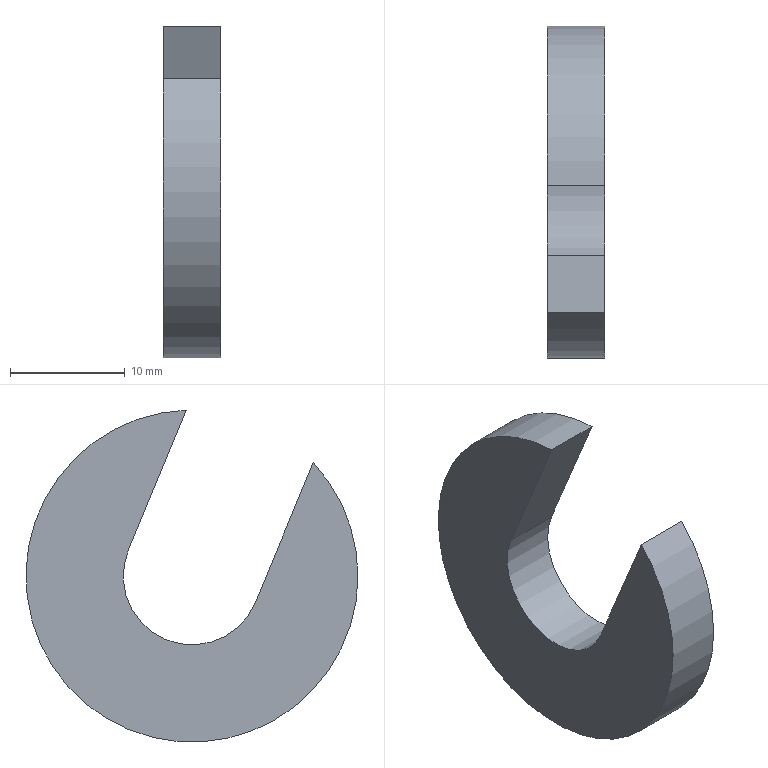Component | NX | WASHER | 1 solid | 6 faces | box 5 x 29 x 28.99 mm | volume 2175 mm3 | plane 4 | cylinder 2 | commonest cylinder face diameters 29 x1 12 x1
STEP:
#1=CARTESIAN_POINT('',(0.,0.,0.));
#2=DIRECTION('',(0.,0.,1.));
#3=DIRECTION('',(1.,0.,0.));
#4=AXIS2_PLACEMENT_3D('',#1,#2,#3);
#5=CARTESIAN_POINT('',(40.592,68.075,199.554));
#6=VERTEX_POINT('',#5);
#7=CARTESIAN_POINT('',(40.592,63.035,211.754));
#8=VERTEX_POINT('',#7);
#9=CARTESIAN_POINT('',(40.592,68.075,199.554));
#10=DIRECTION('',(0.,-0.3818,0.9242));
#11=VECTOR('',#10,1.);
#12=LINE('',#9,#11);
#13=CARTESIAN_POINT('',(45.592,68.075,199.554));
#14=DIRECTION('',(0.,-0.9242,-0.3818));
#15=DIRECTION('',(1.,0.,0.));
#16=AXIS2_PLACEMENT_3D('',#13,#14,#15);
#17=PLANE('',#16);
#18=CARTESIAN_POINT('',(-5.,0.));
#19=DIRECTION('',(0.,1.));
#20=VECTOR('',#19,1.);
#21=LINE('',#18,#20);
#22=(GEOMETRIC_REPRESENTATION_CONTEXT(2)PARAMETRIC_REPRESENTATION_CONTEXT()REPRESENTATION_CONTEXT('',''));
#23=DEFINITIONAL_REPRESENTATION('',(#21),#22);
#24=PCURVE('',#17,#23);
#25=CARTESIAN_POINT('',(40.592,73.621,201.845));
#26=DIRECTION('',(1.,0.,0.));
#27=DIRECTION('',(0.,0.9242,0.3818));
#28=AXIS2_PLACEMENT_3D('',#25,#26,#27);
#29=PLANE('',#28);
#30=CARTESIAN_POINT('',(-6.,-0.));
#31=DIRECTION('',(0.,1.));
#32=VECTOR('',#31,1.);
#33=LINE('',#30,#32);
#34=(GEOMETRIC_REPRESENTATION_CONTEXT(2)PARAMETRIC_REPRESENTATION_CONTEXT()REPRESENTATION_CONTEXT('',''));
#35=DEFINITIONAL_REPRESENTATION('',(#33),#34);
#36=PCURVE('',#29,#35);
#37=SURFACE_CURVE('',#12,(#24,#36),.PCURVE_S1.);
#38=EDGE_CURVE('',#6,#8,#37,.T.);
#39=ORIENTED_EDGE('',*,*,#38,.T.);
#40=CARTESIAN_POINT('',(45.592,63.035,211.754));
#41=VERTEX_POINT('',#40);
#42=CARTESIAN_POINT('',(45.592,63.035,211.754));
#43=DIRECTION('',(-1.,0.,0.));
#44=VECTOR('',#43,1.);
#45=LINE('',#42,#44);
#46=CARTESIAN_POINT('',(0.,13.2));
#47=DIRECTION('',(-1.,0.));
#48=VECTOR('',#47,1.);
#49=LINE('',#46,#48);
#50=(GEOMETRIC_REPRESENTATION_CONTEXT(2)PARAMETRIC_REPRESENTATION_CONTEXT()REPRESENTATION_CONTEXT('',''));
#51=DEFINITIONAL_REPRESENTATION('',(#49),#50);
#52=PCURVE('',#17,#51);
#53=CARTESIAN_POINT('',(45.592,73.621,201.845));
#54=DIRECTION('',(-1.,0.,0.));
#55=DIRECTION('',(0.,-0.9242,-0.3818));
#56=AXIS2_PLACEMENT_3D('',#53,#54,#55);
#57=CYLINDRICAL_SURFACE('',#56,14.5);
#58=CARTESIAN_POINT('',(7.427,0.));
#59=DIRECTION('',(0.,1.));
#60=VECTOR('',#59,1.);
#61=LINE('',#58,#60);
#62=(GEOMETRIC_REPRESENTATION_CONTEXT(2)PARAMETRIC_REPRESENTATION_CONTEXT()REPRESENTATION_CONTEXT('',''));
#63=DEFINITIONAL_REPRESENTATION('',(#61),#62);
#64=PCURVE('',#57,#63);
#65=SURFACE_CURVE('',#45,(#52,#64),.PCURVE_S1.);
#66=EDGE_CURVE('',#41,#8,#65,.T.);
#67=ORIENTED_EDGE('',*,*,#66,.F.);
#68=CARTESIAN_POINT('',(45.592,68.075,199.554));
#69=VERTEX_POINT('',#68);
#70=CARTESIAN_POINT('',(45.592,68.075,199.554));
#71=DIRECTION('',(0.,-0.3818,0.9242));
#72=VECTOR('',#71,1.);
#73=LINE('',#70,#72);
#74=CARTESIAN_POINT('',(0.,0.));
#75=DIRECTION('',(0.,1.));
#76=VECTOR('',#75,1.);
#77=LINE('',#74,#76);
#78=(GEOMETRIC_REPRESENTATION_CONTEXT(2)PARAMETRIC_REPRESENTATION_CONTEXT()REPRESENTATION_CONTEXT('',''));
#79=DEFINITIONAL_REPRESENTATION('',(#77),#78);
#80=PCURVE('',#17,#79);
#81=CARTESIAN_POINT('',(45.592,73.621,201.845));
#82=DIRECTION('',(1.,0.,0.));
#83=DIRECTION('',(0.,0.9242,0.3818));
#84=AXIS2_PLACEMENT_3D('',#81,#82,#83);
#85=PLANE('',#84);
#86=CARTESIAN_POINT('',(-6.,-0.));
#87=DIRECTION('',(0.,1.));
#88=VECTOR('',#87,1.);
#89=LINE('',#86,#88);
#90=(GEOMETRIC_REPRESENTATION_CONTEXT(2)PARAMETRIC_REPRESENTATION_CONTEXT()REPRESENTATION_CONTEXT('',''));
#91=DEFINITIONAL_REPRESENTATION('',(#89),#90);
#92=PCURVE('',#85,#91);
#93=SURFACE_CURVE('',#73,(#80,#92),.PCURVE_S1.);
#94=EDGE_CURVE('',#69,#41,#93,.T.);
#95=ORIENTED_EDGE('',*,*,#94,.F.);
#96=CARTESIAN_POINT('',(45.592,68.075,199.554));
#97=DIRECTION('',(-1.,0.,0.));
#98=VECTOR('',#97,1.);
#99=LINE('',#96,#98);
#100=CARTESIAN_POINT('',(0.,0.));
#101=DIRECTION('',(-1.,0.));
#102=VECTOR('',#101,1.);
#103=LINE('',#100,#102);
#104=(GEOMETRIC_REPRESENTATION_CONTEXT(2)PARAMETRIC_REPRESENTATION_CONTEXT()REPRESENTATION_CONTEXT('',''));
#105=DEFINITIONAL_REPRESENTATION('',(#103),#104);
#106=PCURVE('',#17,#105);
#107=CARTESIAN_POINT('',(45.592,73.621,201.845));
#108=DIRECTION('',(-1.,0.,0.));
#109=DIRECTION('',(0.,-0.9242,-0.3818));
#110=AXIS2_PLACEMENT_3D('',#107,#108,#109);
#111=CYLINDRICAL_SURFACE('',#110,6.);
#112=CARTESIAN_POINT('',(6.283,0.));
#113=DIRECTION('',(0.,1.));
#114=VECTOR('',#113,1.);
#115=LINE('',#112,#114);
#116=(GEOMETRIC_REPRESENTATION_CONTEXT(2)PARAMETRIC_REPRESENTATION_CONTEXT()REPRESENTATION_CONTEXT('',''));
#117=DEFINITIONAL_REPRESENTATION('',(#115),#116);
#118=PCURVE('',#111,#117);
#119=SURFACE_CURVE('',#99,(#106,#118),.PCURVE_S1.);
#120=EDGE_CURVE('',#69,#6,#119,.T.);
#121=ORIENTED_EDGE('',*,*,#120,.T.);
#122=EDGE_LOOP('',(#39,#67,#95,#121));
#123=FACE_BOUND('',#122,.T.);
#124=ADVANCED_FACE('',(#123),#17,.F.);
#125=CARTESIAN_POINT('',(40.592,74.125,216.336));
#126=VERTEX_POINT('',#125);
#127=CARTESIAN_POINT('',(40.592,73.621,201.845));
#128=DIRECTION('',(1.,0.,0.));
#129=DIRECTION('',(0.,0.9242,0.3818));
#130=AXIS2_PLACEMENT_3D('',#127,#128,#129);
#131=CIRCLE('',#130,14.5);
#132=CARTESIAN_POINT('',(9.425,5.));
#133=DIRECTION('',(-1.,0.));
#134=VECTOR('',#133,1.);
#135=LINE('',#132,#134);
#136=(GEOMETRIC_REPRESENTATION_CONTEXT(2)PARAMETRIC_REPRESENTATION_CONTEXT()REPRESENTATION_CONTEXT('',''));
#137=DEFINITIONAL_REPRESENTATION('',(#135),#136);
#138=PCURVE('',#57,#137);
#139=CARTESIAN_POINT('',(0.,0.));
#140=DIRECTION('',(1.,-0.));
#141=AXIS2_PLACEMENT_2D('',#139,#140);
#142=CIRCLE('',#141,14.5);
#143=(GEOMETRIC_REPRESENTATION_CONTEXT(2)PARAMETRIC_REPRESENTATION_CONTEXT()REPRESENTATION_CONTEXT('',''));
#144=DEFINITIONAL_REPRESENTATION('',(#142),#143);
#145=PCURVE('',#29,#144);
#146=SURFACE_CURVE('',#131,(#138,#145),.PCURVE_S1.);
#147=EDGE_CURVE('',#8,#126,#146,.T.);
#148=ORIENTED_EDGE('',*,*,#147,.T.);
#149=CARTESIAN_POINT('',(45.592,74.125,216.336));
#150=VERTEX_POINT('',#149);
#151=CARTESIAN_POINT('',(45.592,74.125,216.336));
#152=DIRECTION('',(-1.,0.,0.));
#153=VECTOR('',#152,1.);
#154=LINE('',#151,#153);
#155=CARTESIAN_POINT('',(1.997,0.));
#156=DIRECTION('',(0.,1.));
#157=VECTOR('',#156,1.);
#158=LINE('',#155,#157);
#159=(GEOMETRIC_REPRESENTATION_CONTEXT(2)PARAMETRIC_REPRESENTATION_CONTEXT()REPRESENTATION_CONTEXT('',''));
#160=DEFINITIONAL_REPRESENTATION('',(#158),#159);
#161=PCURVE('',#57,#160);
#162=CARTESIAN_POINT('',(45.592,74.125,216.336));
#163=DIRECTION('',(0.,0.9242,0.3818));
#164=DIRECTION('',(-1.,0.,0.));
#165=AXIS2_PLACEMENT_3D('',#162,#163,#164);
#166=PLANE('',#165);
#167=CARTESIAN_POINT('',(0.,0.));
#168=DIRECTION('',(1.,0.));
#169=VECTOR('',#168,1.);
#170=LINE('',#167,#169);
#171=(GEOMETRIC_REPRESENTATION_CONTEXT(2)PARAMETRIC_REPRESENTATION_CONTEXT()REPRESENTATION_CONTEXT('',''));
#172=DEFINITIONAL_REPRESENTATION('',(#170),#171);
#173=PCURVE('',#166,#172);
#174=SURFACE_CURVE('',#154,(#161,#173),.PCURVE_S1.);
#175=EDGE_CURVE('',#150,#126,#174,.T.);
#176=ORIENTED_EDGE('',*,*,#175,.F.);
#177=CARTESIAN_POINT('',(45.592,73.621,201.845));
#178=DIRECTION('',(1.,0.,0.));
#179=DIRECTION('',(0.,0.9242,0.3818));
#180=AXIS2_PLACEMENT_3D('',#177,#178,#179);
#181=CIRCLE('',#180,14.5);
#182=CARTESIAN_POINT('',(9.425,0.));
#183=DIRECTION('',(-1.,0.));
#184=VECTOR('',#183,1.);
#185=LINE('',#182,#184);
#186=(GEOMETRIC_REPRESENTATION_CONTEXT(2)PARAMETRIC_REPRESENTATION_CONTEXT()REPRESENTATION_CONTEXT('',''));
#187=DEFINITIONAL_REPRESENTATION('',(#185),#186);
#188=PCURVE('',#57,#187);
#189=CARTESIAN_POINT('',(0.,0.));
#190=DIRECTION('',(1.,-0.));
#191=AXIS2_PLACEMENT_2D('',#189,#190);
#192=CIRCLE('',#191,14.5);
#193=(GEOMETRIC_REPRESENTATION_CONTEXT(2)PARAMETRIC_REPRESENTATION_CONTEXT()REPRESENTATION_CONTEXT('',''));
#194=DEFINITIONAL_REPRESENTATION('',(#192),#193);
#195=PCURVE('',#85,#194);
#196=SURFACE_CURVE('',#181,(#188,#195),.PCURVE_S1.);
#197=EDGE_CURVE('',#41,#150,#196,.T.);
#198=ORIENTED_EDGE('',*,*,#197,.F.);
#199=ORIENTED_EDGE('',*,*,#66,.T.);
#200=EDGE_LOOP('',(#148,#176,#198,#199));
#201=FACE_BOUND('',#200,.T.);
#202=ADVANCED_FACE('',(#201),#57,.T.);
#203=CARTESIAN_POINT('',(40.592,79.166,204.136));
#204=VERTEX_POINT('',#203);
#205=CARTESIAN_POINT('',(40.592,74.125,216.336));
#206=DIRECTION('',(0.,0.3818,-0.9242));
#207=VECTOR('',#206,1.);
#208=LINE('',#205,#207);
#209=CARTESIAN_POINT('',(5.,0.));
#210=DIRECTION('',(0.,-1.));
#211=VECTOR('',#210,1.);
#212=LINE('',#209,#211);
#213=(GEOMETRIC_REPRESENTATION_CONTEXT(2)PARAMETRIC_REPRESENTATION_CONTEXT()REPRESENTATION_CONTEXT('',''));
#214=DEFINITIONAL_REPRESENTATION('',(#212),#213);
#215=PCURVE('',#166,#214);
#216=CARTESIAN_POINT('',(6.,13.2));
#217=DIRECTION('',(-0.,-1.));
#218=VECTOR('',#217,1.);
#219=LINE('',#216,#218);
#220=(GEOMETRIC_REPRESENTATION_CONTEXT(2)PARAMETRIC_REPRESENTATION_CONTEXT()REPRESENTATION_CONTEXT('',''));
#221=DEFINITIONAL_REPRESENTATION('',(#219),#220);
#222=PCURVE('',#29,#221);
#223=SURFACE_CURVE('',#208,(#215,#222),.PCURVE_S1.);
#224=EDGE_CURVE('',#126,#204,#223,.T.);
#225=ORIENTED_EDGE('',*,*,#224,.T.);
#226=CARTESIAN_POINT('',(45.592,79.166,204.136));
#227=VERTEX_POINT('',#226);
#228=CARTESIAN_POINT('',(45.592,79.166,204.136));
#229=DIRECTION('',(-1.,0.,0.));
#230=VECTOR('',#229,1.);
#231=LINE('',#228,#230);
#232=CARTESIAN_POINT('',(0.,-13.2));
#233=DIRECTION('',(1.,0.));
#234=VECTOR('',#233,1.);
#235=LINE('',#232,#234);
#236=(GEOMETRIC_REPRESENTATION_CONTEXT(2)PARAMETRIC_REPRESENTATION_CONTEXT()REPRESENTATION_CONTEXT('',''));
#237=DEFINITIONAL_REPRESENTATION('',(#235),#236);
#238=PCURVE('',#166,#237);
#239=CARTESIAN_POINT('',(3.142,0.));
#240=DIRECTION('',(0.,1.));
#241=VECTOR('',#240,1.);
#242=LINE('',#239,#241);
#243=(GEOMETRIC_REPRESENTATION_CONTEXT(2)PARAMETRIC_REPRESENTATION_CONTEXT()REPRESENTATION_CONTEXT('',''));
#244=DEFINITIONAL_REPRESENTATION('',(#242),#243);
#245=PCURVE('',#111,#244);
#246=SURFACE_CURVE('',#231,(#238,#245),.PCURVE_S1.);
#247=EDGE_CURVE('',#227,#204,#246,.T.);
#248=ORIENTED_EDGE('',*,*,#247,.F.);
#249=CARTESIAN_POINT('',(45.592,74.125,216.336));
#250=DIRECTION('',(0.,0.3818,-0.9242));
#251=VECTOR('',#250,1.);
#252=LINE('',#249,#251);
#253=CARTESIAN_POINT('',(0.,0.));
#254=DIRECTION('',(0.,-1.));
#255=VECTOR('',#254,1.);
#256=LINE('',#253,#255);
#257=(GEOMETRIC_REPRESENTATION_CONTEXT(2)PARAMETRIC_REPRESENTATION_CONTEXT()REPRESENTATION_CONTEXT('',''));
#258=DEFINITIONAL_REPRESENTATION('',(#256),#257);
#259=PCURVE('',#166,#258);
#260=CARTESIAN_POINT('',(6.,13.2));
#261=DIRECTION('',(-0.,-1.));
#262=VECTOR('',#261,1.);
#263=LINE('',#260,#262);
#264=(GEOMETRIC_REPRESENTATION_CONTEXT(2)PARAMETRIC_REPRESENTATION_CONTEXT()REPRESENTATION_CONTEXT('',''));
#265=DEFINITIONAL_REPRESENTATION('',(#263),#264);
#266=PCURVE('',#85,#265);
#267=SURFACE_CURVE('',#252,(#259,#266),.PCURVE_S1.);
#268=EDGE_CURVE('',#150,#227,#267,.T.);
#269=ORIENTED_EDGE('',*,*,#268,.F.);
#270=ORIENTED_EDGE('',*,*,#175,.T.);
#271=EDGE_LOOP('',(#225,#248,#269,#270));
#272=FACE_BOUND('',#271,.T.);
#273=ADVANCED_FACE('',(#272),#166,.F.);
#274=ORIENTED_EDGE('',*,*,#247,.F.);
#275=CARTESIAN_POINT('',(45.592,73.621,201.845));
#276=DIRECTION('',(-1.,0.,0.));
#277=DIRECTION('',(0.,0.9242,0.3818));
#278=AXIS2_PLACEMENT_3D('',#275,#276,#277);
#279=CIRCLE('',#278,6.);
#280=CARTESIAN_POINT('',(3.142,0.));
#281=DIRECTION('',(1.,0.));
#282=VECTOR('',#281,1.);
#283=LINE('',#280,#282);
#284=(GEOMETRIC_REPRESENTATION_CONTEXT(2)PARAMETRIC_REPRESENTATION_CONTEXT()REPRESENTATION_CONTEXT('',''));
#285=DEFINITIONAL_REPRESENTATION('',(#283),#284);
#286=PCURVE('',#111,#285);
#287=CARTESIAN_POINT('',(6.,0.));
#288=CARTESIAN_POINT('',(6.,-10.392));
#289=CARTESIAN_POINT('',(-3.,-5.196));
#290=CARTESIAN_POINT('',(-12.,-0.));
#291=CARTESIAN_POINT('',(-3.,5.196));
#292=CARTESIAN_POINT('',(6.,10.392));
#293=CARTESIAN_POINT('',(6.,0.));
#294=(BOUNDED_CURVE()B_SPLINE_CURVE(2,(#287,#288,#289,#290,#291,#292,#293),.UNSPECIFIED.,.T.,.F.)B_SPLINE_CURVE_WITH_KNOTS((1,2,2,2,2,1),(-2.094,0.,2.094,4.189,6.283,8.378),.UNSPECIFIED.)CURVE()GEOMETRIC_REPRESENTATION_ITEM()RATIONAL_B_SPLINE_CURVE((1.,0.5,1.,0.5,1.,0.5,1.))REPRESENTATION_ITEM(''));
#295=(GEOMETRIC_REPRESENTATION_CONTEXT(2)PARAMETRIC_REPRESENTATION_CONTEXT()REPRESENTATION_CONTEXT('',''));
#296=DEFINITIONAL_REPRESENTATION('',(#294),#295);
#297=PCURVE('',#85,#296);
#298=SURFACE_CURVE('',#279,(#286,#297),.PCURVE_S1.);
#299=EDGE_CURVE('',#227,#69,#298,.T.);
#300=ORIENTED_EDGE('',*,*,#299,.T.);
#301=ORIENTED_EDGE('',*,*,#120,.T.);
#302=CARTESIAN_POINT('',(40.592,73.621,201.845));
#303=DIRECTION('',(-1.,0.,0.));
#304=DIRECTION('',(0.,0.9242,0.3818));
#305=AXIS2_PLACEMENT_3D('',#302,#303,#304);
#306=CIRCLE('',#305,6.);
#307=CARTESIAN_POINT('',(3.142,5.));
#308=DIRECTION('',(1.,0.));
#309=VECTOR('',#308,1.);
#310=LINE('',#307,#309);
#311=(GEOMETRIC_REPRESENTATION_CONTEXT(2)PARAMETRIC_REPRESENTATION_CONTEXT()REPRESENTATION_CONTEXT('',''));
#312=DEFINITIONAL_REPRESENTATION('',(#310),#311);
#313=PCURVE('',#111,#312);
#314=CARTESIAN_POINT('',(6.,0.));
#315=CARTESIAN_POINT('',(6.,-10.392));
#316=CARTESIAN_POINT('',(-3.,-5.196));
#317=CARTESIAN_POINT('',(-12.,-0.));
#318=CARTESIAN_POINT('',(-3.,5.196));
#319=CARTESIAN_POINT('',(6.,10.392));
#320=CARTESIAN_POINT('',(6.,0.));
#321=(BOUNDED_CURVE()B_SPLINE_CURVE(2,(#314,#315,#316,#317,#318,#319,#320),.UNSPECIFIED.,.T.,.F.)B_SPLINE_CURVE_WITH_KNOTS((1,2,2,2,2,1),(-2.094,0.,2.094,4.189,6.283,8.378),.UNSPECIFIED.)CURVE()GEOMETRIC_REPRESENTATION_ITEM()RATIONAL_B_SPLINE_CURVE((1.,0.5,1.,0.5,1.,0.5,1.))REPRESENTATION_ITEM(''));
#322=(GEOMETRIC_REPRESENTATION_CONTEXT(2)PARAMETRIC_REPRESENTATION_CONTEXT()REPRESENTATION_CONTEXT('',''));
#323=DEFINITIONAL_REPRESENTATION('',(#321),#322);
#324=PCURVE('',#29,#323);
#325=SURFACE_CURVE('',#306,(#313,#324),.PCURVE_S1.);
#326=EDGE_CURVE('',#204,#6,#325,.T.);
#327=ORIENTED_EDGE('',*,*,#326,.F.);
#328=EDGE_LOOP('',(#274,#300,#301,#327));
#329=FACE_BOUND('',#328,.F.);
#330=ADVANCED_FACE('',(#329),#111,.F.);
#331=ORIENTED_EDGE('',*,*,#94,.T.);
#332=ORIENTED_EDGE('',*,*,#197,.T.);
#333=ORIENTED_EDGE('',*,*,#268,.T.);
#334=ORIENTED_EDGE('',*,*,#299,.T.);
#335=EDGE_LOOP('',(#331,#332,#333,#334));
#336=FACE_BOUND('',#335,.T.);
#337=ADVANCED_FACE('',(#336),#85,.T.);
#338=ORIENTED_EDGE('',*,*,#38,.F.);
#339=ORIENTED_EDGE('',*,*,#326,.F.);
#340=ORIENTED_EDGE('',*,*,#224,.F.);
#341=ORIENTED_EDGE('',*,*,#147,.F.);
#342=EDGE_LOOP('',(#338,#339,#340,#341));
#343=FACE_BOUND('',#342,.T.);
#344=ADVANCED_FACE('',(#343),#29,.F.);
#345=CLOSED_SHELL('',(#124,#202,#273,#330,#337,#344));
#346=MANIFOLD_SOLID_BREP('',#345);
#347=(LENGTH_UNIT()NAMED_UNIT(*)SI_UNIT(.MILLI.,.METRE.));
#348=UNCERTAINTY_MEASURE_WITH_UNIT(LENGTH_MEASURE(0.0000001),#347,'','');
#349=(NAMED_UNIT(*)PLANE_ANGLE_UNIT()SI_UNIT($,.RADIAN.));
#350=(NAMED_UNIT(*)SI_UNIT($,.STERADIAN.)SOLID_ANGLE_UNIT());
#351=(GEOMETRIC_REPRESENTATION_CONTEXT(3)GLOBAL_UNCERTAINTY_ASSIGNED_CONTEXT((#348))GLOBAL_UNIT_ASSIGNED_CONTEXT((#347,#349,#350))REPRESENTATION_CONTEXT('',''));
#352=ADVANCED_BREP_SHAPE_REPRESENTATION('',(#4,#346),#351);